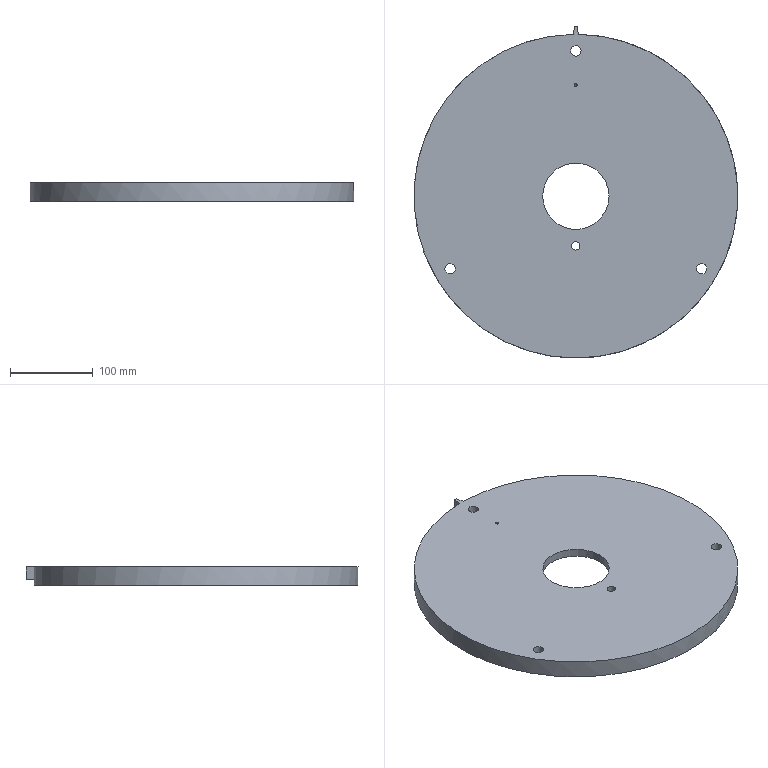Component | NX | DRIVINGFLANGE | 1 solid | 17 faces | volume 1994956 mm3 | cylinder 9 | plane 7 | torus 1 | commonest cylinder face diameters 12.5 x3 240 x1 390 x1 80 x1 10 x1 3 x1 410.011 x1